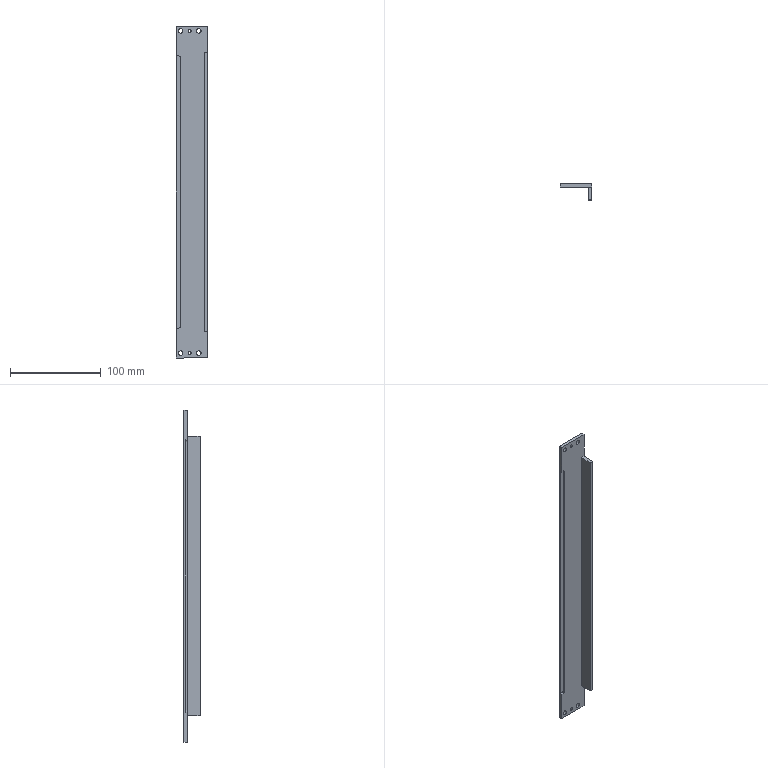Component | SolidWorks | CTM-HVS-52-OA-02-14-1 | 1 solid | 28 faces | box 35 x 18 x 366 mm | volume 65111 mm3 | cylinder 14 | plane 14 | commonest cylinder face diameters 5 x10 3.3 x4 | material 316L
build123d program:
from build123d import *

# Parameters (mm, degrees)
SKETCH1_W                  = 366
SKETCH1_H                  = 35
EXTRUDE1_DEPTH             = 4
SKETCH2_W                  = 308
SKETCH2_H                  = 4
EXTRUDE2_DEPTH             = 14
SKETCH4_W                  = 300
SKETCH4_H                  = 5
CUT_EXTRUDE1_DEPTH         = 2
FILLET1_R                  = 2.5
M6_TAPPED_HOLE1_AT_2_COUNT = 2
M6_TAPPED_HOLE1_AT_2_PITCH = 20


with BuildPart() as part:
    # Sketch1 → Extrude1 (new body)
    with BuildSketch(Plane.XY):
        Rectangle(SKETCH1_W, SKETCH1_H)
    extrude(amount=EXTRUDE1_DEPTH)

    # Sketch2 → Extrude2 (add)
    with BuildSketch(Plane.XY.offset(4)):
        with Locations((0, -15.5)):
            Rectangle(SKETCH2_W, SKETCH2_H)
    extrude(amount=EXTRUDE2_DEPTH)

    # Sketch4 → Cut-Extrude1 (cut)
    with BuildSketch(Plane.XY.offset(4)):
        with Locations((0, 15)):
            Rectangle(SKETCH4_W, SKETCH4_H)
    extrude(amount=-CUT_EXTRUDE1_DEPTH, mode=Mode.SUBTRACT)

    # Fillet1
    fillet1_edges = [part.edges().sort_by_distance(p)[0] for p in [
        (-150, 12.5, 3),
        (150, 12.5, 3),
    ]]
    fillet(fillet1_edges, radius=FILLET1_R)

    # Sketch5 → M6 Tapped Hole1 (revolve, cut)
    with BuildSketch(Plane(origin=(-177.5, 12.5, 4), x_dir=(0, -1, 0), z_dir=(1, 0, 0))):
        Polygon((0, 0), (0, 18.502), (2.5, 17), (2.5, 0), align=None)
    m6_tapped_hole1 = revolve(axis=Axis((-177.5, 12.5, 10.35), (0, 0, -1)), mode=Mode.SUBTRACT)

    # M6 Tapped Hole1 at 2: M6 Tapped Hole1 ×2
    with Locations(*[(0, -i * M6_TAPPED_HOLE1_AT_2_PITCH, 0) for i in range(1, M6_TAPPED_HOLE1_AT_2_COUNT)]):
        add(m6_tapped_hole1, mode=Mode.SUBTRACT)

    # Sketch7 → M4 Tapped Hole1 (revolve, cut)
    with BuildSketch(Plane(origin=(-177.5, 2.5, 4), x_dir=(0, -1, 0), z_dir=(1, 0, 0))):
        Polygon((0, 0), (0, 12.491), (1.65, 11.5), (1.65, 0), align=None)
    m4_tapped_hole1 = revolve(axis=Axis((-177.5, 2.5, 10.35), (0, 0, -1)), mode=Mode.SUBTRACT)

    # Mirror1: M6 Tapped Hole1, M4 Tapped Hole1 across plane
    add(m6_tapped_hole1.mirror(Plane(origin=(0, 0, 0), x_dir=(0, 0, 1), z_dir=(1, 0, 0))), mode=Mode.SUBTRACT)
    add(m4_tapped_hole1.mirror(Plane(origin=(0, 0, 0), x_dir=(0, 0, 1), z_dir=(1, 0, 0))), mode=Mode.SUBTRACT)

    # Mirror1 copy 1 sketch → Mirror1 copy 1 (revolve, cut)
    with BuildSketch(Plane(origin=(177.5, -7.5, 4), x_dir=(0, -1, 0), z_dir=(-1, 0, 0))):
        Polygon((0, 0), (0, -18.502), (2.5, -17), (2.5, 0), align=None)
    revolve(axis=Axis((177.5, -7.5, 10.35), (0, 0, 1)), mode=Mode.SUBTRACT)


solid = part.part

# Placed as in the assembly
solid = solid.moved(Location((292.693, -60.557, 192.5), (90, 0, 90)))
STEP:
#1=COLOUR_RGB('',0.7922,0.8196,0.9333);
#2=FILL_AREA_STYLE_COLOUR('',#1);
#3=FILL_AREA_STYLE('',(#2));
#4=SURFACE_STYLE_FILL_AREA(#3);
#5=SURFACE_SIDE_STYLE('',(#4));
#6=SURFACE_STYLE_USAGE(.BOTH.,#5);
#7=PRESENTATION_STYLE_ASSIGNMENT((#6));
#8=CARTESIAN_POINT('',(11.425,-2.384,14.502));
#9=VERTEX_POINT('',#8);
#10=CARTESIAN_POINT('',(11.425,-2.384,14.632));
#11=VERTEX_POINT('',#10);
#12=CARTESIAN_POINT('',(11.425,-2.384,14.567));
#13=DIRECTION('',(-0.,-1.,-0.));
#14=DIRECTION('',(0.,0.,1.));
#15=AXIS2_PLACEMENT_3D('',#12,#13,#14);
#16=CIRCLE('',#15,0.06496);
#17=EDGE_CURVE('',#9,#11,#16,.T.);
#18=ORIENTED_EDGE('',*,*,#17,.F.);
#19=CARTESIAN_POINT('',(11.425,-2.542,14.502));
#20=VERTEX_POINT('',#19);
#21=CARTESIAN_POINT('',(11.425,-2.542,14.502));
#22=DIRECTION('',(-0.,-1.,-0.));
#23=VECTOR('',#22,39.37);
#24=LINE('',#21,#23);
#25=EDGE_CURVE('',#9,#20,#24,.T.);
#26=ORIENTED_EDGE('',*,*,#25,.T.);
#27=CARTESIAN_POINT('',(11.425,-2.542,14.632));
#28=VERTEX_POINT('',#27);
#29=CARTESIAN_POINT('',(11.425,-2.542,14.567));
#30=DIRECTION('',(-0.,-1.,-0.));
#31=DIRECTION('',(0.,0.,1.));
#32=AXIS2_PLACEMENT_3D('',#29,#30,#31);
#33=CIRCLE('',#32,0.06496);
#34=EDGE_CURVE('',#20,#28,#33,.T.);
#35=ORIENTED_EDGE('',*,*,#34,.T.);
#36=CARTESIAN_POINT('',(11.425,-2.542,14.632));
#37=DIRECTION('',(-0.,-1.,-0.));
#38=VECTOR('',#37,39.37);
#39=LINE('',#36,#38);
#40=EDGE_CURVE('',#11,#28,#39,.T.);
#41=ORIENTED_EDGE('',*,*,#40,.F.);
#42=EDGE_LOOP('',(#18,#26,#35,#41));
#43=FACE_OUTER_BOUND('',#42,.T.);
#44=CARTESIAN_POINT('',(11.425,-2.542,14.567));
#45=DIRECTION('',(-0.,-1.,-0.));
#46=DIRECTION('',(0.,0.,1.));
#47=AXIS2_PLACEMENT_3D('',#44,#45,#46);
#48=CYLINDRICAL_SURFACE('',#47,0.06496);
#49=ADVANCED_FACE('',(#43),#48,.F.);
#50=CARTESIAN_POINT('',(11.031,-2.384,14.469));
#51=VERTEX_POINT('',#50);
#52=CARTESIAN_POINT('',(11.031,-2.384,14.665));
#53=VERTEX_POINT('',#52);
#54=CARTESIAN_POINT('',(11.031,-2.384,14.567));
#55=DIRECTION('',(-0.,-1.,-0.));
#56=DIRECTION('',(0.,0.,1.));
#57=AXIS2_PLACEMENT_3D('',#54,#55,#56);
#58=CIRCLE('',#57,0.09843);
#59=EDGE_CURVE('',#51,#53,#58,.T.);
#60=ORIENTED_EDGE('',*,*,#59,.F.);
#61=CARTESIAN_POINT('',(11.031,-2.542,14.469));
#62=VERTEX_POINT('',#61);
#63=CARTESIAN_POINT('',(11.031,-2.542,14.469));
#64=DIRECTION('',(-0.,-1.,-0.));
#65=VECTOR('',#64,39.37);
#66=LINE('',#63,#65);
#67=EDGE_CURVE('',#51,#62,#66,.T.);
#68=ORIENTED_EDGE('',*,*,#67,.T.);
#69=CARTESIAN_POINT('',(11.031,-2.542,14.665));
#70=VERTEX_POINT('',#69);
#71=CARTESIAN_POINT('',(11.031,-2.542,14.567));
#72=DIRECTION('',(-0.,-1.,-0.));
#73=DIRECTION('',(0.,0.,1.));
#74=AXIS2_PLACEMENT_3D('',#71,#72,#73);
#75=CIRCLE('',#74,0.09843);
#76=EDGE_CURVE('',#62,#70,#75,.T.);
#77=ORIENTED_EDGE('',*,*,#76,.T.);
#78=CARTESIAN_POINT('',(11.031,-2.542,14.665));
#79=DIRECTION('',(-0.,-1.,-0.));
#80=VECTOR('',#79,39.37);
#81=LINE('',#78,#80);
#82=EDGE_CURVE('',#53,#70,#81,.T.);
#83=ORIENTED_EDGE('',*,*,#82,.F.);
#84=EDGE_LOOP('',(#60,#68,#77,#83));
#85=FACE_OUTER_BOUND('',#84,.T.);
#86=CARTESIAN_POINT('',(11.031,-2.542,14.567));
#87=DIRECTION('',(-0.,-1.,-0.));
#88=DIRECTION('',(0.,0.,1.));
#89=AXIS2_PLACEMENT_3D('',#86,#87,#88);
#90=CYLINDRICAL_SURFACE('',#89,0.09843);
#91=ADVANCED_FACE('',(#85),#90,.F.);
#92=CARTESIAN_POINT('',(11.819,-2.384,14.469));
#93=VERTEX_POINT('',#92);
#94=CARTESIAN_POINT('',(11.819,-2.384,14.665));
#95=VERTEX_POINT('',#94);
#96=CARTESIAN_POINT('',(11.819,-2.384,14.567));
#97=DIRECTION('',(-0.,-1.,-0.));
#98=DIRECTION('',(0.,0.,1.));
#99=AXIS2_PLACEMENT_3D('',#96,#97,#98);
#100=CIRCLE('',#99,0.09843);
#101=EDGE_CURVE('',#93,#95,#100,.T.);
#102=ORIENTED_EDGE('',*,*,#101,.F.);
#103=CARTESIAN_POINT('',(11.819,-2.542,14.469));
#104=VERTEX_POINT('',#103);
#105=CARTESIAN_POINT('',(11.819,-2.542,14.469));
#106=DIRECTION('',(-0.,-1.,-0.));
#107=VECTOR('',#106,39.37);
#108=LINE('',#105,#107);
#109=EDGE_CURVE('',#93,#104,#108,.T.);
#110=ORIENTED_EDGE('',*,*,#109,.T.);
#111=CARTESIAN_POINT('',(11.819,-2.542,14.665));
#112=VERTEX_POINT('',#111);
#113=CARTESIAN_POINT('',(11.819,-2.542,14.567));
#114=DIRECTION('',(-0.,-1.,-0.));
#115=DIRECTION('',(0.,0.,1.));
#116=AXIS2_PLACEMENT_3D('',#113,#114,#115);
#117=CIRCLE('',#116,0.09843);
#118=EDGE_CURVE('',#104,#112,#117,.T.);
#119=ORIENTED_EDGE('',*,*,#118,.T.);
#120=CARTESIAN_POINT('',(11.819,-2.542,14.665));
#121=DIRECTION('',(-0.,-1.,-0.));
#122=VECTOR('',#121,39.37);
#123=LINE('',#120,#122);
#124=EDGE_CURVE('',#95,#112,#123,.T.);
#125=ORIENTED_EDGE('',*,*,#124,.F.);
#126=EDGE_LOOP('',(#102,#110,#119,#125));
#127=FACE_OUTER_BOUND('',#126,.T.);
#128=CARTESIAN_POINT('',(11.819,-2.542,14.567));
#129=DIRECTION('',(-0.,-1.,-0.));
#130=DIRECTION('',(0.,0.,1.));
#131=AXIS2_PLACEMENT_3D('',#128,#129,#130);
#132=CYLINDRICAL_SURFACE('',#131,0.09843);
#133=ADVANCED_FACE('',(#127),#132,.F.);
#134=CARTESIAN_POINT('',(11.425,-2.384,0.5256));
#135=VERTEX_POINT('',#134);
#136=CARTESIAN_POINT('',(11.425,-2.384,0.6555));
#137=VERTEX_POINT('',#136);
#138=CARTESIAN_POINT('',(11.425,-2.384,0.5906));
#139=DIRECTION('',(-0.,-1.,-0.));
#140=DIRECTION('',(0.,0.,1.));
#141=AXIS2_PLACEMENT_3D('',#138,#139,#140);
#142=CIRCLE('',#141,0.06496);
#143=EDGE_CURVE('',#135,#137,#142,.T.);
#144=ORIENTED_EDGE('',*,*,#143,.F.);
#145=CARTESIAN_POINT('',(11.425,-2.542,0.5256));
#146=VERTEX_POINT('',#145);
#147=CARTESIAN_POINT('',(11.425,-2.542,0.5256));
#148=DIRECTION('',(-0.,-1.,-0.));
#149=VECTOR('',#148,39.37);
#150=LINE('',#147,#149);
#151=EDGE_CURVE('',#135,#146,#150,.T.);
#152=ORIENTED_EDGE('',*,*,#151,.T.);
#153=CARTESIAN_POINT('',(11.425,-2.542,0.6555));
#154=VERTEX_POINT('',#153);
#155=CARTESIAN_POINT('',(11.425,-2.542,0.5906));
#156=DIRECTION('',(-0.,-1.,-0.));
#157=DIRECTION('',(0.,0.,1.));
#158=AXIS2_PLACEMENT_3D('',#155,#156,#157);
#159=CIRCLE('',#158,0.06496);
#160=EDGE_CURVE('',#146,#154,#159,.T.);
#161=ORIENTED_EDGE('',*,*,#160,.T.);
#162=CARTESIAN_POINT('',(11.425,-2.542,0.6555));
#163=DIRECTION('',(-0.,-1.,-0.));
#164=VECTOR('',#163,39.37);
#165=LINE('',#162,#164);
#166=EDGE_CURVE('',#137,#154,#165,.T.);
#167=ORIENTED_EDGE('',*,*,#166,.F.);
#168=EDGE_LOOP('',(#144,#152,#161,#167));
#169=FACE_OUTER_BOUND('',#168,.T.);
#170=CARTESIAN_POINT('',(11.425,-2.542,0.5906));
#171=DIRECTION('',(-0.,-1.,-0.));
#172=DIRECTION('',(0.,0.,1.));
#173=AXIS2_PLACEMENT_3D('',#170,#171,#172);
#174=CYLINDRICAL_SURFACE('',#173,0.06496);
#175=ADVANCED_FACE('',(#169),#174,.F.);
#176=CARTESIAN_POINT('',(11.031,-2.384,0.4921));
#177=VERTEX_POINT('',#176);
#178=CARTESIAN_POINT('',(11.031,-2.384,0.689));
#179=VERTEX_POINT('',#178);
#180=CARTESIAN_POINT('',(11.031,-2.384,0.5906));
#181=DIRECTION('',(-0.,-1.,-0.));
#182=DIRECTION('',(0.,0.,1.));
#183=AXIS2_PLACEMENT_3D('',#180,#181,#182);
#184=CIRCLE('',#183,0.09843);
#185=EDGE_CURVE('',#177,#179,#184,.T.);
#186=ORIENTED_EDGE('',*,*,#185,.F.);
#187=CARTESIAN_POINT('',(11.031,-2.542,0.4921));
#188=VERTEX_POINT('',#187);
#189=CARTESIAN_POINT('',(11.031,-2.542,0.4921));
#190=DIRECTION('',(-0.,-1.,-0.));
#191=VECTOR('',#190,39.37);
#192=LINE('',#189,#191);
#193=EDGE_CURVE('',#177,#188,#192,.T.);
#194=ORIENTED_EDGE('',*,*,#193,.T.);
#195=CARTESIAN_POINT('',(11.031,-2.542,0.689));
#196=VERTEX_POINT('',#195);
#197=CARTESIAN_POINT('',(11.031,-2.542,0.5906));
#198=DIRECTION('',(-0.,-1.,-0.));
#199=DIRECTION('',(0.,0.,1.));
#200=AXIS2_PLACEMENT_3D('',#197,#198,#199);
#201=CIRCLE('',#200,0.09843);
#202=EDGE_CURVE('',#188,#196,#201,.T.);
#203=ORIENTED_EDGE('',*,*,#202,.T.);
#204=CARTESIAN_POINT('',(11.031,-2.542,0.689));
#205=DIRECTION('',(-0.,-1.,-0.));
#206=VECTOR('',#205,39.37);
#207=LINE('',#204,#206);
#208=EDGE_CURVE('',#179,#196,#207,.T.);
#209=ORIENTED_EDGE('',*,*,#208,.F.);
#210=EDGE_LOOP('',(#186,#194,#203,#209));
#211=FACE_OUTER_BOUND('',#210,.T.);
#212=CARTESIAN_POINT('',(11.031,-2.542,0.5906));
#213=DIRECTION('',(-0.,-1.,-0.));
#214=DIRECTION('',(0.,0.,1.));
#215=AXIS2_PLACEMENT_3D('',#212,#213,#214);
#216=CYLINDRICAL_SURFACE('',#215,0.09843);
#217=ADVANCED_FACE('',(#211),#216,.F.);
#218=CARTESIAN_POINT('',(11.819,-2.384,0.4921));
#219=VERTEX_POINT('',#218);
#220=CARTESIAN_POINT('',(11.819,-2.384,0.689));
#221=VERTEX_POINT('',#220);
#222=CARTESIAN_POINT('',(11.819,-2.384,0.5906));
#223=DIRECTION('',(-0.,-1.,-0.));
#224=DIRECTION('',(0.,0.,1.));
#225=AXIS2_PLACEMENT_3D('',#222,#223,#224);
#226=CIRCLE('',#225,0.09843);
#227=EDGE_CURVE('',#219,#221,#226,.T.);
#228=ORIENTED_EDGE('',*,*,#227,.F.);
#229=CARTESIAN_POINT('',(11.819,-2.542,0.4921));
#230=VERTEX_POINT('',#229);
#231=CARTESIAN_POINT('',(11.819,-2.542,0.4921));
#232=DIRECTION('',(-0.,-1.,-0.));
#233=VECTOR('',#232,39.37);
#234=LINE('',#231,#233);
#235=EDGE_CURVE('',#219,#230,#234,.T.);
#236=ORIENTED_EDGE('',*,*,#235,.T.);
#237=CARTESIAN_POINT('',(11.819,-2.542,0.689));
#238=VERTEX_POINT('',#237);
#239=CARTESIAN_POINT('',(11.819,-2.542,0.5906));
#240=DIRECTION('',(-0.,-1.,-0.));
#241=DIRECTION('',(0.,0.,1.));
#242=AXIS2_PLACEMENT_3D('',#239,#240,#241);
#243=CIRCLE('',#242,0.09843);
#244=EDGE_CURVE('',#230,#238,#243,.T.);
#245=ORIENTED_EDGE('',*,*,#244,.T.);
#246=CARTESIAN_POINT('',(11.819,-2.542,0.689));
#247=DIRECTION('',(-0.,-1.,-0.));
#248=VECTOR('',#247,39.37);
#249=LINE('',#246,#248);
#250=EDGE_CURVE('',#221,#238,#249,.T.);
#251=ORIENTED_EDGE('',*,*,#250,.F.);
#252=EDGE_LOOP('',(#228,#236,#245,#251));
#253=FACE_OUTER_BOUND('',#252,.T.);
#254=CARTESIAN_POINT('',(11.819,-2.542,0.5906));
#255=DIRECTION('',(-0.,-1.,-0.));
#256=DIRECTION('',(0.,0.,1.));
#257=AXIS2_PLACEMENT_3D('',#254,#255,#256);
#258=CYLINDRICAL_SURFACE('',#257,0.09843);
#259=ADVANCED_FACE('',(#253),#258,.F.);
#260=CARTESIAN_POINT('',(12.212,-2.384,14.783));
#261=VERTEX_POINT('',#260);
#262=CARTESIAN_POINT('',(10.834,-2.384,14.783));
#263=VERTEX_POINT('',#262);
#264=CARTESIAN_POINT('',(10.834,-2.384,14.783));
#265=DIRECTION('',(-1.,0.,-0.));
#266=VECTOR('',#265,39.37);
#267=LINE('',#264,#266);
#268=EDGE_CURVE('',#261,#263,#267,.T.);
#269=ORIENTED_EDGE('',*,*,#268,.T.);
#270=CARTESIAN_POINT('',(10.834,-2.542,14.783));
#271=VERTEX_POINT('',#270);
#272=CARTESIAN_POINT('',(10.834,-2.542,14.783));
#273=DIRECTION('',(0.,1.,0.));
#274=VECTOR('',#273,39.37);
#275=LINE('',#272,#274);
#276=EDGE_CURVE('',#271,#263,#275,.T.);
#277=ORIENTED_EDGE('',*,*,#276,.F.);
#278=CARTESIAN_POINT('',(12.212,-2.542,14.783));
#279=VERTEX_POINT('',#278);
#280=CARTESIAN_POINT('',(10.834,-2.542,14.783));
#281=DIRECTION('',(-1.,0.,-0.));
#282=VECTOR('',#281,39.37);
#283=LINE('',#280,#282);
#284=EDGE_CURVE('',#279,#271,#283,.T.);
#285=ORIENTED_EDGE('',*,*,#284,.F.);
#286=CARTESIAN_POINT('',(12.212,-2.542,14.783));
#287=DIRECTION('',(0.,1.,0.));
#288=VECTOR('',#287,39.37);
#289=LINE('',#286,#288);
#290=EDGE_CURVE('',#279,#261,#289,.T.);
#291=ORIENTED_EDGE('',*,*,#290,.T.);
#292=EDGE_LOOP('',(#269,#277,#285,#291));
#293=FACE_OUTER_BOUND('',#292,.T.);
#294=CARTESIAN_POINT('',(10.834,-2.542,14.783));
#295=DIRECTION('',(0.,0.,-1.));
#296=DIRECTION('',(-0.,-1.,-0.));
#297=AXIS2_PLACEMENT_3D('',#294,#295,#296);
#298=PLANE('',#297);
#299=ADVANCED_FACE('',(#293),#298,.F.);
#300=CARTESIAN_POINT('',(10.834,-2.542,1.673));
#301=VERTEX_POINT('',#300);
#302=CARTESIAN_POINT('',(10.834,-2.542,0.374));
#303=VERTEX_POINT('',#302);
#304=CARTESIAN_POINT('',(10.834,-2.542,0.374));
#305=DIRECTION('',(0.,-0.,-1.));
#306=VECTOR('',#305,39.37);
#307=LINE('',#304,#306);
#308=EDGE_CURVE('',#301,#303,#307,.T.);
#309=ORIENTED_EDGE('',*,*,#308,.F.);
#310=CARTESIAN_POINT('',(10.834,-2.463,1.673));
#311=VERTEX_POINT('',#310);
#312=CARTESIAN_POINT('',(10.834,-2.463,1.673));
#313=DIRECTION('',(-0.,-1.,-0.));
#314=VECTOR('',#313,39.37);
#315=LINE('',#312,#314);
#316=EDGE_CURVE('',#311,#301,#315,.T.);
#317=ORIENTED_EDGE('',*,*,#316,.F.);
#318=CARTESIAN_POINT('',(10.834,-2.463,13.484));
#319=VERTEX_POINT('',#318);
#320=CARTESIAN_POINT('',(10.834,-2.463,13.484));
#321=DIRECTION('',(0.,-0.,-1.));
#322=VECTOR('',#321,39.37);
#323=LINE('',#320,#322);
#324=EDGE_CURVE('',#319,#311,#323,.T.);
#325=ORIENTED_EDGE('',*,*,#324,.F.);
#326=CARTESIAN_POINT('',(10.834,-2.542,13.484));
#327=VERTEX_POINT('',#326);
#328=CARTESIAN_POINT('',(10.834,-2.463,13.484));
#329=DIRECTION('',(-0.,-1.,-0.));
#330=VECTOR('',#329,39.37);
#331=LINE('',#328,#330);
#332=EDGE_CURVE('',#319,#327,#331,.T.);
#333=ORIENTED_EDGE('',*,*,#332,.T.);
#334=CARTESIAN_POINT('',(10.834,-2.542,0.374));
#335=DIRECTION('',(0.,-0.,-1.));
#336=VECTOR('',#335,39.37);
#337=LINE('',#334,#336);
#338=EDGE_CURVE('',#271,#327,#337,.T.);
#339=ORIENTED_EDGE('',*,*,#338,.F.);
#340=ORIENTED_EDGE('',*,*,#276,.T.);
#341=CARTESIAN_POINT('',(10.834,-2.384,0.374));
#342=VERTEX_POINT('',#341);
#343=CARTESIAN_POINT('',(10.834,-2.384,0.374));
#344=DIRECTION('',(0.,-0.,-1.));
#345=VECTOR('',#344,39.37);
#346=LINE('',#343,#345);
#347=EDGE_CURVE('',#263,#342,#346,.T.);
#348=ORIENTED_EDGE('',*,*,#347,.T.);
#349=CARTESIAN_POINT('',(10.834,-2.542,0.374));
#350=DIRECTION('',(0.,1.,0.));
#351=VECTOR('',#350,39.37);
#352=LINE('',#349,#351);
#353=EDGE_CURVE('',#303,#342,#352,.T.);
#354=ORIENTED_EDGE('',*,*,#353,.F.);
#355=EDGE_LOOP('',(#309,#317,#325,#333,#339,#340,#348,#354));
#356=FACE_OUTER_BOUND('',#355,.T.);
#357=CARTESIAN_POINT('',(10.834,-2.542,0.374));
#358=DIRECTION('',(1.,-0.,0.));
#359=DIRECTION('',(0.,1.,0.));
#360=AXIS2_PLACEMENT_3D('',#357,#358,#359);
#361=PLANE('',#360);
#362=ADVANCED_FACE('',(#356),#361,.F.);
#363=CARTESIAN_POINT('',(12.212,-2.384,0.374));
#364=VERTEX_POINT('',#363);
#365=CARTESIAN_POINT('',(10.834,-2.384,0.374));
#366=DIRECTION('',(1.,-0.,0.));
#367=VECTOR('',#366,39.37);
#368=LINE('',#365,#367);
#369=EDGE_CURVE('',#342,#364,#368,.T.);
#370=ORIENTED_EDGE('',*,*,#369,.T.);
#371=CARTESIAN_POINT('',(12.212,-2.542,0.374));
#372=VERTEX_POINT('',#371);
#373=CARTESIAN_POINT('',(12.212,-2.542,0.374));
#374=DIRECTION('',(0.,1.,0.));
#375=VECTOR('',#374,39.37);
#376=LINE('',#373,#375);
#377=EDGE_CURVE('',#372,#364,#376,.T.);
#378=ORIENTED_EDGE('',*,*,#377,.F.);
#379=CARTESIAN_POINT('',(10.834,-2.542,0.374));
#380=DIRECTION('',(1.,-0.,0.));
#381=VECTOR('',#380,39.37);
#382=LINE('',#379,#381);
#383=EDGE_CURVE('',#303,#372,#382,.T.);
#384=ORIENTED_EDGE('',*,*,#383,.F.);
#385=ORIENTED_EDGE('',*,*,#353,.T.);
#386=EDGE_LOOP('',(#370,#378,#384,#385));
#387=FACE_OUTER_BOUND('',#386,.T.);
#388=CARTESIAN_POINT('',(10.834,-2.542,0.374));
#389=DIRECTION('',(-0.,-0.,1.));
#390=DIRECTION('',(0.,1.,0.));
#391=AXIS2_PLACEMENT_3D('',#388,#389,#390);
#392=PLANE('',#391);
#393=ADVANCED_FACE('',(#387),#392,.F.);
#394=CARTESIAN_POINT('',(12.212,-2.384,0.374));
#395=DIRECTION('',(-0.,0.,1.));
#396=VECTOR('',#395,39.37);
#397=LINE('',#394,#396);
#398=EDGE_CURVE('',#364,#261,#397,.T.);
#399=ORIENTED_EDGE('',*,*,#398,.T.);
#400=ORIENTED_EDGE('',*,*,#290,.F.);
#401=CARTESIAN_POINT('',(12.212,-2.542,13.642));
#402=VERTEX_POINT('',#401);
#403=CARTESIAN_POINT('',(12.212,-2.542,0.374));
#404=DIRECTION('',(-0.,0.,1.));
#405=VECTOR('',#404,39.37);
#406=LINE('',#403,#405);
#407=EDGE_CURVE('',#402,#279,#406,.T.);
#408=ORIENTED_EDGE('',*,*,#407,.F.);
#409=CARTESIAN_POINT('',(12.212,-3.093,13.642));
#410=VERTEX_POINT('',#409);
#411=CARTESIAN_POINT('',(12.212,-3.093,13.642));
#412=DIRECTION('',(0.,1.,0.));
#413=VECTOR('',#412,39.37);
#414=LINE('',#411,#413);
#415=EDGE_CURVE('',#410,#402,#414,.T.);
#416=ORIENTED_EDGE('',*,*,#415,.F.);
#417=CARTESIAN_POINT('',(12.212,-3.093,1.516));
#418=VERTEX_POINT('',#417);
#419=CARTESIAN_POINT('',(12.212,-3.093,1.516));
#420=DIRECTION('',(-0.,0.,1.));
#421=VECTOR('',#420,39.37);
#422=LINE('',#419,#421);
#423=EDGE_CURVE('',#418,#410,#422,.T.);
#424=ORIENTED_EDGE('',*,*,#423,.F.);
#425=CARTESIAN_POINT('',(12.212,-2.542,1.516));
#426=VERTEX_POINT('',#425);
#427=CARTESIAN_POINT('',(12.212,-3.093,1.516));
#428=DIRECTION('',(0.,1.,0.));
#429=VECTOR('',#428,39.37);
#430=LINE('',#427,#429);
#431=EDGE_CURVE('',#418,#426,#430,.T.);
#432=ORIENTED_EDGE('',*,*,#431,.T.);
#433=CARTESIAN_POINT('',(12.212,-2.542,0.374));
#434=DIRECTION('',(-0.,0.,1.));
#435=VECTOR('',#434,39.37);
#436=LINE('',#433,#435);
#437=EDGE_CURVE('',#372,#426,#436,.T.);
#438=ORIENTED_EDGE('',*,*,#437,.F.);
#439=ORIENTED_EDGE('',*,*,#377,.T.);
#440=EDGE_LOOP('',(#399,#400,#408,#416,#424,#432,#438,#439));
#441=FACE_OUTER_BOUND('',#440,.T.);
#442=CARTESIAN_POINT('',(12.212,-2.542,0.374));
#443=DIRECTION('',(-1.,0.,-0.));
#444=DIRECTION('',(-0.,-1.,-0.));
#445=AXIS2_PLACEMENT_3D('',#442,#443,#444);
#446=PLANE('',#445);
#447=ADVANCED_FACE('',(#441),#446,.F.);
#448=CARTESIAN_POINT('',(11.425,-2.542,14.567));
#449=DIRECTION('',(-0.,-1.,-0.));
#450=DIRECTION('',(0.,0.,1.));
#451=AXIS2_PLACEMENT_3D('',#448,#449,#450);
#452=CIRCLE('',#451,0.06496);
#453=EDGE_CURVE('',#28,#20,#452,.T.);
#454=ORIENTED_EDGE('',*,*,#453,.F.);
#455=ORIENTED_EDGE('',*,*,#34,.F.);
#456=EDGE_LOOP('',(#454,#455));
#457=FACE_BOUND('',#456,.T.);
#458=CARTESIAN_POINT('',(11.031,-2.542,14.567));
#459=DIRECTION('',(-0.,-1.,-0.));
#460=DIRECTION('',(0.,0.,1.));
#461=AXIS2_PLACEMENT_3D('',#458,#459,#460);
#462=CIRCLE('',#461,0.09843);
#463=EDGE_CURVE('',#70,#62,#462,.T.);
#464=ORIENTED_EDGE('',*,*,#463,.F.);
#465=ORIENTED_EDGE('',*,*,#76,.F.);
#466=EDGE_LOOP('',(#464,#465));
#467=FACE_BOUND('',#466,.T.);
#468=CARTESIAN_POINT('',(11.819,-2.542,14.567));
#469=DIRECTION('',(-0.,-1.,-0.));
#470=DIRECTION('',(0.,0.,1.));
#471=AXIS2_PLACEMENT_3D('',#468,#469,#470);
#472=CIRCLE('',#471,0.09843);
#473=EDGE_CURVE('',#112,#104,#472,.T.);
#474=ORIENTED_EDGE('',*,*,#473,.F.);
#475=ORIENTED_EDGE('',*,*,#118,.F.);
#476=EDGE_LOOP('',(#474,#475));
#477=FACE_BOUND('',#476,.T.);
#478=CARTESIAN_POINT('',(11.425,-2.542,0.5906));
#479=DIRECTION('',(-0.,-1.,-0.));
#480=DIRECTION('',(0.,0.,1.));
#481=AXIS2_PLACEMENT_3D('',#478,#479,#480);
#482=CIRCLE('',#481,0.06496);
#483=EDGE_CURVE('',#154,#146,#482,.T.);
#484=ORIENTED_EDGE('',*,*,#483,.F.);
#485=ORIENTED_EDGE('',*,*,#160,.F.);
#486=EDGE_LOOP('',(#484,#485));
#487=FACE_BOUND('',#486,.T.);
#488=CARTESIAN_POINT('',(11.031,-2.542,0.5906));
#489=DIRECTION('',(-0.,-1.,-0.));
#490=DIRECTION('',(0.,0.,1.));
#491=AXIS2_PLACEMENT_3D('',#488,#489,#490);
#492=CIRCLE('',#491,0.09843);
#493=EDGE_CURVE('',#196,#188,#492,.T.);
#494=ORIENTED_EDGE('',*,*,#493,.F.);
#495=ORIENTED_EDGE('',*,*,#202,.F.);
#496=EDGE_LOOP('',(#494,#495));
#497=FACE_BOUND('',#496,.T.);
#498=CARTESIAN_POINT('',(11.819,-2.542,0.5906));
#499=DIRECTION('',(-0.,-1.,-0.));
#500=DIRECTION('',(0.,0.,1.));
#501=AXIS2_PLACEMENT_3D('',#498,#499,#500);
#502=CIRCLE('',#501,0.09843);
#503=EDGE_CURVE('',#238,#230,#502,.T.);
#504=ORIENTED_EDGE('',*,*,#503,.F.);
#505=ORIENTED_EDGE('',*,*,#244,.F.);
#506=EDGE_LOOP('',(#504,#505));
#507=FACE_BOUND('',#506,.T.);
#508=CARTESIAN_POINT('',(10.933,-2.542,1.673));
#509=VERTEX_POINT('',#508);
#510=CARTESIAN_POINT('',(11.031,-2.542,1.673));
#511=DIRECTION('',(1.,-0.,0.));
#512=VECTOR('',#511,39.37);
#513=LINE('',#510,#512);
#514=EDGE_CURVE('',#301,#509,#513,.T.);
#515=ORIENTED_EDGE('',*,*,#514,.F.);
#516=ORIENTED_EDGE('',*,*,#308,.T.);
#517=ORIENTED_EDGE('',*,*,#383,.T.);
#518=ORIENTED_EDGE('',*,*,#437,.T.);
#519=CARTESIAN_POINT('',(12.055,-2.542,1.516));
#520=VERTEX_POINT('',#519);
#521=CARTESIAN_POINT('',(12.055,-2.542,1.516));
#522=DIRECTION('',(1.,-0.,0.));
#523=VECTOR('',#522,39.37);
#524=LINE('',#521,#523);
#525=EDGE_CURVE('',#520,#426,#524,.T.);
#526=ORIENTED_EDGE('',*,*,#525,.F.);
#527=CARTESIAN_POINT('',(12.055,-2.542,13.642));
#528=VERTEX_POINT('',#527);
#529=CARTESIAN_POINT('',(12.055,-2.542,1.516));
#530=DIRECTION('',(0.,-0.,-1.));
#531=VECTOR('',#530,39.37);
#532=LINE('',#529,#531);
#533=EDGE_CURVE('',#528,#520,#532,.T.);
#534=ORIENTED_EDGE('',*,*,#533,.F.);
#535=CARTESIAN_POINT('',(12.055,-2.542,13.642));
#536=DIRECTION('',(-1.,0.,-0.));
#537=VECTOR('',#536,39.37);
#538=LINE('',#535,#537);
#539=EDGE_CURVE('',#402,#528,#538,.T.);
#540=ORIENTED_EDGE('',*,*,#539,.F.);
#541=ORIENTED_EDGE('',*,*,#407,.T.);
#542=ORIENTED_EDGE('',*,*,#284,.T.);
#543=ORIENTED_EDGE('',*,*,#338,.T.);
#544=CARTESIAN_POINT('',(10.933,-2.542,13.484));
#545=VERTEX_POINT('',#544);
#546=CARTESIAN_POINT('',(11.031,-2.542,13.484));
#547=DIRECTION('',(-1.,0.,-0.));
#548=VECTOR('',#547,39.37);
#549=LINE('',#546,#548);
#550=EDGE_CURVE('',#545,#327,#549,.T.);
#551=ORIENTED_EDGE('',*,*,#550,.F.);
#552=CARTESIAN_POINT('',(11.031,-2.542,13.386));
#553=VERTEX_POINT('',#552);
#554=CARTESIAN_POINT('',(10.933,-2.542,13.386));
#555=DIRECTION('',(0.,1.,0.));
#556=DIRECTION('',(0.,0.,1.));
#557=AXIS2_PLACEMENT_3D('',#554,#555,#556);
#558=CIRCLE('',#557,0.09843);
#559=EDGE_CURVE('',#545,#553,#558,.T.);
#560=ORIENTED_EDGE('',*,*,#559,.T.);
#561=CARTESIAN_POINT('',(11.031,-2.542,1.772));
#562=VERTEX_POINT('',#561);
#563=CARTESIAN_POINT('',(11.031,-2.542,13.484));
#564=DIRECTION('',(-0.,0.,1.));
#565=VECTOR('',#564,39.37);
#566=LINE('',#563,#565);
#567=EDGE_CURVE('',#562,#553,#566,.T.);
#568=ORIENTED_EDGE('',*,*,#567,.F.);
#569=CARTESIAN_POINT('',(10.933,-2.542,1.772));
#570=DIRECTION('',(0.,1.,0.));
#571=DIRECTION('',(0.,0.,1.));
#572=AXIS2_PLACEMENT_3D('',#569,#570,#571);
#573=CIRCLE('',#572,0.09843);
#574=EDGE_CURVE('',#562,#509,#573,.T.);
#575=ORIENTED_EDGE('',*,*,#574,.T.);
#576=EDGE_LOOP('',(#515,#516,#517,#518,#526,#534,#540,#541,#542,#543,#551,#560,#568,#575));
#577=FACE_OUTER_BOUND('',#576,.T.);
#578=CARTESIAN_POINT('',(12.212,-2.542,14.783));
#579=DIRECTION('',(-0.,-1.,-0.));
#580=DIRECTION('',(-0.,0.,1.));
#581=AXIS2_PLACEMENT_3D('',#578,#579,#580);
#582=PLANE('',#581);
#583=ADVANCED_FACE('',(#457,#467,#477,#487,#497,#507,#577),#582,.T.);
#584=CARTESIAN_POINT('',(11.425,-2.384,14.567));
#585=DIRECTION('',(-0.,-1.,-0.));
#586=DIRECTION('',(0.,0.,1.));
#587=AXIS2_PLACEMENT_3D('',#584,#585,#586);
#588=CIRCLE('',#587,0.06496);
#589=EDGE_CURVE('',#11,#9,#588,.T.);
#590=ORIENTED_EDGE('',*,*,#589,.T.);
#591=ORIENTED_EDGE('',*,*,#17,.T.);
#592=EDGE_LOOP('',(#590,#591));
#593=FACE_BOUND('',#592,.T.);
#594=CARTESIAN_POINT('',(11.031,-2.384,14.567));
#595=DIRECTION('',(-0.,-1.,-0.));
#596=DIRECTION('',(0.,0.,1.));
#597=AXIS2_PLACEMENT_3D('',#594,#595,#596);
#598=CIRCLE('',#597,0.09843);
#599=EDGE_CURVE('',#53,#51,#598,.T.);
#600=ORIENTED_EDGE('',*,*,#599,.T.);
#601=ORIENTED_EDGE('',*,*,#59,.T.);
#602=EDGE_LOOP('',(#600,#601));
#603=FACE_BOUND('',#602,.T.);
#604=CARTESIAN_POINT('',(11.819,-2.384,14.567));
#605=DIRECTION('',(-0.,-1.,-0.));
#606=DIRECTION('',(0.,0.,1.));
#607=AXIS2_PLACEMENT_3D('',#604,#605,#606);
#608=CIRCLE('',#607,0.09843);
#609=EDGE_CURVE('',#95,#93,#608,.T.);
#610=ORIENTED_EDGE('',*,*,#609,.T.);
#611=ORIENTED_EDGE('',*,*,#101,.T.);
#612=EDGE_LOOP('',(#610,#611));
#613=FACE_BOUND('',#612,.T.);
#614=CARTESIAN_POINT('',(11.425,-2.384,0.5906));
#615=DIRECTION('',(-0.,-1.,-0.));
#616=DIRECTION('',(0.,0.,1.));
#617=AXIS2_PLACEMENT_3D('',#614,#615,#616);
#618=CIRCLE('',#617,0.06496);
#619=EDGE_CURVE('',#137,#135,#618,.T.);
#620=ORIENTED_EDGE('',*,*,#619,.T.);
#621=ORIENTED_EDGE('',*,*,#143,.T.);
#622=EDGE_LOOP('',(#620,#621));
#623=FACE_BOUND('',#622,.T.);
#624=CARTESIAN_POINT('',(11.031,-2.384,0.5906));
#625=DIRECTION('',(-0.,-1.,-0.));
#626=DIRECTION('',(0.,0.,1.));
#627=AXIS2_PLACEMENT_3D('',#624,#625,#626);
#628=CIRCLE('',#627,0.09843);
#629=EDGE_CURVE('',#179,#177,#628,.T.);
#630=ORIENTED_EDGE('',*,*,#629,.T.);
#631=ORIENTED_EDGE('',*,*,#185,.T.);
#632=EDGE_LOOP('',(#630,#631));
#633=FACE_BOUND('',#632,.T.);
#634=CARTESIAN_POINT('',(11.819,-2.384,0.5906));
#635=DIRECTION('',(-0.,-1.,-0.));
#636=DIRECTION('',(0.,0.,1.));
#637=AXIS2_PLACEMENT_3D('',#634,#635,#636);
#638=CIRCLE('',#637,0.09843);
#639=EDGE_CURVE('',#221,#219,#638,.T.);
#640=ORIENTED_EDGE('',*,*,#639,.T.);
#641=ORIENTED_EDGE('',*,*,#227,.T.);
#642=EDGE_LOOP('',(#640,#641));
#643=FACE_BOUND('',#642,.T.);
#644=ORIENTED_EDGE('',*,*,#268,.F.);
#645=ORIENTED_EDGE('',*,*,#398,.F.);
#646=ORIENTED_EDGE('',*,*,#369,.F.);
#647=ORIENTED_EDGE('',*,*,#347,.F.);
#648=EDGE_LOOP('',(#644,#645,#646,#647));
#649=FACE_OUTER_BOUND('',#648,.T.);
#650=CARTESIAN_POINT('',(12.212,-2.384,14.783));
#651=DIRECTION('',(-0.,-1.,-0.));
#652=DIRECTION('',(-0.,0.,1.));
#653=AXIS2_PLACEMENT_3D('',#650,#651,#652);
#654=PLANE('',#653);
#655=ADVANCED_FACE('',(#593,#603,#613,#623,#633,#643,#649),#654,.F.);
#656=ORIENTED_EDGE('',*,*,#539,.T.);
#657=CARTESIAN_POINT('',(12.055,-3.093,13.642));
#658=VERTEX_POINT('',#657);
#659=CARTESIAN_POINT('',(12.055,-3.093,13.642));
#660=DIRECTION('',(0.,1.,0.));
#661=VECTOR('',#660,39.37);
#662=LINE('',#659,#661);
#663=EDGE_CURVE('',#658,#528,#662,.T.);
#664=ORIENTED_EDGE('',*,*,#663,.F.);
#665=CARTESIAN_POINT('',(12.055,-3.093,13.642));
#666=DIRECTION('',(-1.,0.,-0.));
#667=VECTOR('',#666,39.37);
#668=LINE('',#665,#667);
#669=EDGE_CURVE('',#410,#658,#668,.T.);
#670=ORIENTED_EDGE('',*,*,#669,.F.);
#671=ORIENTED_EDGE('',*,*,#415,.T.);
#672=EDGE_LOOP('',(#656,#664,#670,#671));
#673=FACE_OUTER_BOUND('',#672,.T.);
#674=CARTESIAN_POINT('',(12.055,-3.093,13.642));
#675=DIRECTION('',(0.,0.,-1.));
#676=DIRECTION('',(-0.,-1.,-0.));
#677=AXIS2_PLACEMENT_3D('',#674,#675,#676);
#678=PLANE('',#677);
#679=ADVANCED_FACE('',(#673),#678,.F.);
#680=ORIENTED_EDGE('',*,*,#533,.T.);
#681=CARTESIAN_POINT('',(12.055,-3.093,1.516));
#682=VERTEX_POINT('',#681);
#683=CARTESIAN_POINT('',(12.055,-3.093,1.516));
#684=DIRECTION('',(0.,1.,0.));
#685=VECTOR('',#684,39.37);
#686=LINE('',#683,#685);
#687=EDGE_CURVE('',#682,#520,#686,.T.);
#688=ORIENTED_EDGE('',*,*,#687,.F.);
#689=CARTESIAN_POINT('',(12.055,-3.093,1.516));
#690=DIRECTION('',(0.,-0.,-1.));
#691=VECTOR('',#690,39.37);
#692=LINE('',#689,#691);
#693=EDGE_CURVE('',#658,#682,#692,.T.);
#694=ORIENTED_EDGE('',*,*,#693,.F.);
#695=ORIENTED_EDGE('',*,*,#663,.T.);
#696=EDGE_LOOP('',(#680,#688,#694,#695));
#697=FACE_OUTER_BOUND('',#696,.T.);
#698=CARTESIAN_POINT('',(12.055,-3.093,1.516));
#699=DIRECTION('',(1.,-0.,0.));
#700=DIRECTION('',(0.,1.,0.));
#701=AXIS2_PLACEMENT_3D('',#698,#699,#700);
#702=PLANE('',#701);
#703=ADVANCED_FACE('',(#697),#702,.F.);
#704=ORIENTED_EDGE('',*,*,#525,.T.);
#705=ORIENTED_EDGE('',*,*,#431,.F.);
#706=CARTESIAN_POINT('',(12.055,-3.093,1.516));
#707=DIRECTION('',(1.,-0.,0.));
#708=VECTOR('',#707,39.37);
#709=LINE('',#706,#708);
#710=EDGE_CURVE('',#682,#418,#709,.T.);
#711=ORIENTED_EDGE('',*,*,#710,.F.);
#712=ORIENTED_EDGE('',*,*,#687,.T.);
#713=EDGE_LOOP('',(#704,#705,#711,#712));
#714=FACE_OUTER_BOUND('',#713,.T.);
#715=CARTESIAN_POINT('',(12.055,-3.093,1.516));
#716=DIRECTION('',(-0.,-0.,1.));
#717=DIRECTION('',(0.,1.,0.));
#718=AXIS2_PLACEMENT_3D('',#715,#716,#717);
#719=PLANE('',#718);
#720=ADVANCED_FACE('',(#714),#719,.F.);
#721=ORIENTED_EDGE('',*,*,#669,.T.);
#722=ORIENTED_EDGE('',*,*,#693,.T.);
#723=ORIENTED_EDGE('',*,*,#710,.T.);
#724=ORIENTED_EDGE('',*,*,#423,.T.);
#725=EDGE_LOOP('',(#721,#722,#723,#724));
#726=FACE_OUTER_BOUND('',#725,.T.);
#727=CARTESIAN_POINT('',(12.212,-3.093,13.642));
#728=DIRECTION('',(-0.,-1.,-0.));
#729=DIRECTION('',(-0.,0.,1.));
#730=AXIS2_PLACEMENT_3D('',#727,#728,#729);
#731=PLANE('',#730);
#732=ADVANCED_FACE('',(#726),#731,.T.);
#733=ORIENTED_EDGE('',*,*,#514,.T.);
#734=CARTESIAN_POINT('',(10.933,-2.463,1.673));
#735=VERTEX_POINT('',#734);
#736=CARTESIAN_POINT('',(10.933,-2.463,1.673));
#737=DIRECTION('',(0.,1.,0.));
#738=VECTOR('',#737,39.37);
#739=LINE('',#736,#738);
#740=EDGE_CURVE('',#509,#735,#739,.T.);
#741=ORIENTED_EDGE('',*,*,#740,.T.);
#742=CARTESIAN_POINT('',(11.031,-2.463,1.673));
#743=DIRECTION('',(1.,-0.,0.));
#744=VECTOR('',#743,39.37);
#745=LINE('',#742,#744);
#746=EDGE_CURVE('',#311,#735,#745,.T.);
#747=ORIENTED_EDGE('',*,*,#746,.F.);
#748=ORIENTED_EDGE('',*,*,#316,.T.);
#749=EDGE_LOOP('',(#733,#741,#747,#748));
#750=FACE_OUTER_BOUND('',#749,.T.);
#751=CARTESIAN_POINT('',(11.031,-2.463,1.673));
#752=DIRECTION('',(0.,0.,-1.));
#753=DIRECTION('',(-0.,-1.,-0.));
#754=AXIS2_PLACEMENT_3D('',#751,#752,#753);
#755=PLANE('',#754);
#756=ADVANCED_FACE('',(#750),#755,.F.);
#757=CARTESIAN_POINT('',(10.933,-2.463,13.484));
#758=VERTEX_POINT('',#757);
#759=CARTESIAN_POINT('',(11.031,-2.463,13.484));
#760=DIRECTION('',(-1.,0.,-0.));
#761=VECTOR('',#760,39.37);
#762=LINE('',#759,#761);
#763=EDGE_CURVE('',#758,#319,#762,.T.);
#764=ORIENTED_EDGE('',*,*,#763,.F.);
#765=CARTESIAN_POINT('',(10.933,-2.542,13.484));
#766=DIRECTION('',(-0.,-1.,-0.));
#767=VECTOR('',#766,39.37);
#768=LINE('',#765,#767);
#769=EDGE_CURVE('',#758,#545,#768,.T.);
#770=ORIENTED_EDGE('',*,*,#769,.T.);
#771=ORIENTED_EDGE('',*,*,#550,.T.);
#772=ORIENTED_EDGE('',*,*,#332,.F.);
#773=EDGE_LOOP('',(#764,#770,#771,#772));
#774=FACE_OUTER_BOUND('',#773,.T.);
#775=CARTESIAN_POINT('',(11.031,-2.463,13.484));
#776=DIRECTION('',(-0.,-0.,1.));
#777=DIRECTION('',(0.,1.,0.));
#778=AXIS2_PLACEMENT_3D('',#775,#776,#777);
#779=PLANE('',#778);
#780=ADVANCED_FACE('',(#774),#779,.F.);
#781=ORIENTED_EDGE('',*,*,#567,.T.);
#782=CARTESIAN_POINT('',(11.031,-2.463,13.386));
#783=VERTEX_POINT('',#782);
#784=CARTESIAN_POINT('',(11.031,-2.463,13.386));
#785=DIRECTION('',(0.,1.,0.));
#786=VECTOR('',#785,39.37);
#787=LINE('',#784,#786);
#788=EDGE_CURVE('',#553,#783,#787,.T.);
#789=ORIENTED_EDGE('',*,*,#788,.T.);
#790=CARTESIAN_POINT('',(11.031,-2.463,1.772));
#791=VERTEX_POINT('',#790);
#792=CARTESIAN_POINT('',(11.031,-2.463,13.484));
#793=DIRECTION('',(-0.,0.,1.));
#794=VECTOR('',#793,39.37);
#795=LINE('',#792,#794);
#796=EDGE_CURVE('',#791,#783,#795,.T.);
#797=ORIENTED_EDGE('',*,*,#796,.F.);
#798=CARTESIAN_POINT('',(11.031,-2.542,1.772));
#799=DIRECTION('',(-0.,-1.,-0.));
#800=VECTOR('',#799,39.37);
#801=LINE('',#798,#800);
#802=EDGE_CURVE('',#791,#562,#801,.T.);
#803=ORIENTED_EDGE('',*,*,#802,.T.);
#804=EDGE_LOOP('',(#781,#789,#797,#803));
#805=FACE_OUTER_BOUND('',#804,.T.);
#806=CARTESIAN_POINT('',(11.031,-2.463,13.484));
#807=DIRECTION('',(1.,-0.,0.));
#808=DIRECTION('',(-0.,0.,1.));
#809=AXIS2_PLACEMENT_3D('',#806,#807,#808);
#810=PLANE('',#809);
#811=ADVANCED_FACE('',(#805),#810,.F.);
#812=ORIENTED_EDGE('',*,*,#796,.T.);
#813=CARTESIAN_POINT('',(10.933,-2.463,13.386));
#814=DIRECTION('',(-0.,-1.,-0.));
#815=DIRECTION('',(0.,0.,1.));
#816=AXIS2_PLACEMENT_3D('',#813,#814,#815);
#817=CIRCLE('',#816,0.09843);
#818=EDGE_CURVE('',#783,#758,#817,.T.);
#819=ORIENTED_EDGE('',*,*,#818,.T.);
#820=ORIENTED_EDGE('',*,*,#763,.T.);
#821=ORIENTED_EDGE('',*,*,#324,.T.);
#822=ORIENTED_EDGE('',*,*,#746,.T.);
#823=CARTESIAN_POINT('',(10.933,-2.463,1.772));
#824=DIRECTION('',(-0.,-1.,-0.));
#825=DIRECTION('',(0.,0.,1.));
#826=AXIS2_PLACEMENT_3D('',#823,#824,#825);
#827=CIRCLE('',#826,0.09843);
#828=EDGE_CURVE('',#735,#791,#827,.T.);
#829=ORIENTED_EDGE('',*,*,#828,.T.);
#830=EDGE_LOOP('',(#812,#819,#820,#821,#822,#829));
#831=FACE_OUTER_BOUND('',#830,.T.);
#832=CARTESIAN_POINT('',(10.834,-2.463,1.673));
#833=DIRECTION('',(-0.,-1.,-0.));
#834=DIRECTION('',(-0.,0.,1.));
#835=AXIS2_PLACEMENT_3D('',#832,#833,#834);
#836=PLANE('',#835);
#837=ADVANCED_FACE('',(#831),#836,.T.);
#838=ORIENTED_EDGE('',*,*,#818,.F.);
#839=ORIENTED_EDGE('',*,*,#788,.F.);
#840=ORIENTED_EDGE('',*,*,#559,.F.);
#841=ORIENTED_EDGE('',*,*,#769,.F.);
#842=EDGE_LOOP('',(#838,#839,#840,#841));
#843=FACE_OUTER_BOUND('',#842,.T.);
#844=CARTESIAN_POINT('',(10.933,-2.463,13.386));
#845=DIRECTION('',(0.,1.,0.));
#846=DIRECTION('',(0.,0.,-1.));
#847=AXIS2_PLACEMENT_3D('',#844,#845,#846);
#848=CYLINDRICAL_SURFACE('',#847,0.09843);
#849=ADVANCED_FACE('',(#843),#848,.F.);
#850=ORIENTED_EDGE('',*,*,#828,.F.);
#851=ORIENTED_EDGE('',*,*,#740,.F.);
#852=ORIENTED_EDGE('',*,*,#574,.F.);
#853=ORIENTED_EDGE('',*,*,#802,.F.);
#854=EDGE_LOOP('',(#850,#851,#852,#853));
#855=FACE_OUTER_BOUND('',#854,.T.);
#856=CARTESIAN_POINT('',(10.933,-2.463,1.772));
#857=DIRECTION('',(0.,1.,0.));
#858=DIRECTION('',(0.,0.,-1.));
#859=AXIS2_PLACEMENT_3D('',#856,#857,#858);
#860=CYLINDRICAL_SURFACE('',#859,0.09843);
#861=ADVANCED_FACE('',(#855),#860,.F.);
#862=ORIENTED_EDGE('',*,*,#235,.F.);
#863=ORIENTED_EDGE('',*,*,#639,.F.);
#864=ORIENTED_EDGE('',*,*,#250,.T.);
#865=ORIENTED_EDGE('',*,*,#503,.T.);
#866=EDGE_LOOP('',(#862,#863,#864,#865));
#867=FACE_OUTER_BOUND('',#866,.T.);
#868=CARTESIAN_POINT('',(11.819,-2.542,0.5906));
#869=DIRECTION('',(-0.,-1.,-0.));
#870=DIRECTION('',(0.,0.,1.));
#871=AXIS2_PLACEMENT_3D('',#868,#869,#870);
#872=CYLINDRICAL_SURFACE('',#871,0.09843);
#873=ADVANCED_FACE('',(#867),#872,.F.);
#874=ORIENTED_EDGE('',*,*,#193,.F.);
#875=ORIENTED_EDGE('',*,*,#629,.F.);
#876=ORIENTED_EDGE('',*,*,#208,.T.);
#877=ORIENTED_EDGE('',*,*,#493,.T.);
#878=EDGE_LOOP('',(#874,#875,#876,#877));
#879=FACE_OUTER_BOUND('',#878,.T.);
#880=CARTESIAN_POINT('',(11.031,-2.542,0.5906));
#881=DIRECTION('',(-0.,-1.,-0.));
#882=DIRECTION('',(0.,0.,1.));
#883=AXIS2_PLACEMENT_3D('',#880,#881,#882);
#884=CYLINDRICAL_SURFACE('',#883,0.09843);
#885=ADVANCED_FACE('',(#879),#884,.F.);
#886=ORIENTED_EDGE('',*,*,#151,.F.);
#887=ORIENTED_EDGE('',*,*,#619,.F.);
#888=ORIENTED_EDGE('',*,*,#166,.T.);
#889=ORIENTED_EDGE('',*,*,#483,.T.);
#890=EDGE_LOOP('',(#886,#887,#888,#889));
#891=FACE_OUTER_BOUND('',#890,.T.);
#892=CARTESIAN_POINT('',(11.425,-2.542,0.5906));
#893=DIRECTION('',(-0.,-1.,-0.));
#894=DIRECTION('',(0.,0.,1.));
#895=AXIS2_PLACEMENT_3D('',#892,#893,#894);
#896=CYLINDRICAL_SURFACE('',#895,0.06496);
#897=ADVANCED_FACE('',(#891),#896,.F.);
#898=ORIENTED_EDGE('',*,*,#109,.F.);
#899=ORIENTED_EDGE('',*,*,#609,.F.);
#900=ORIENTED_EDGE('',*,*,#124,.T.);
#901=ORIENTED_EDGE('',*,*,#473,.T.);
#902=EDGE_LOOP('',(#898,#899,#900,#901));
#903=FACE_OUTER_BOUND('',#902,.T.);
#904=CARTESIAN_POINT('',(11.819,-2.542,14.567));
#905=DIRECTION('',(-0.,-1.,-0.));
#906=DIRECTION('',(0.,0.,1.));
#907=AXIS2_PLACEMENT_3D('',#904,#905,#906);
#908=CYLINDRICAL_SURFACE('',#907,0.09843);
#909=ADVANCED_FACE('',(#903),#908,.F.);
#910=ORIENTED_EDGE('',*,*,#67,.F.);
#911=ORIENTED_EDGE('',*,*,#599,.F.);
#912=ORIENTED_EDGE('',*,*,#82,.T.);
#913=ORIENTED_EDGE('',*,*,#463,.T.);
#914=EDGE_LOOP('',(#910,#911,#912,#913));
#915=FACE_OUTER_BOUND('',#914,.T.);
#916=CARTESIAN_POINT('',(11.031,-2.542,14.567));
#917=DIRECTION('',(-0.,-1.,-0.));
#918=DIRECTION('',(0.,0.,1.));
#919=AXIS2_PLACEMENT_3D('',#916,#917,#918);
#920=CYLINDRICAL_SURFACE('',#919,0.09843);
#921=ADVANCED_FACE('',(#915),#920,.F.);
#922=ORIENTED_EDGE('',*,*,#25,.F.);
#923=ORIENTED_EDGE('',*,*,#589,.F.);
#924=ORIENTED_EDGE('',*,*,#40,.T.);
#925=ORIENTED_EDGE('',*,*,#453,.T.);
#926=EDGE_LOOP('',(#922,#923,#924,#925));
#927=FACE_OUTER_BOUND('',#926,.T.);
#928=CARTESIAN_POINT('',(11.425,-2.542,14.567));
#929=DIRECTION('',(-0.,-1.,-0.));
#930=DIRECTION('',(0.,0.,1.));
#931=AXIS2_PLACEMENT_3D('',#928,#929,#930);
#932=CYLINDRICAL_SURFACE('',#931,0.06496);
#933=ADVANCED_FACE('',(#927),#932,.F.);
#934=CLOSED_SHELL('',(#49,#91,#133,#175,#217,#259,#299,#362,#393,#447,#583,#655,#679,#703,#720,#732,#756,#780,#811,#837,#849,#861,#873,#885,#897,#909,#921,#933));
#935=MANIFOLD_SOLID_BREP('',#934);
#936=STYLED_ITEM('',(#7),#935);
#937=(LENGTH_UNIT()NAMED_UNIT(*)SI_UNIT($,.METRE.));
#938=LENGTH_MEASURE_WITH_UNIT(LENGTH_MEASURE(0.0254),#937);
#939=DIMENSIONAL_EXPONENTS(1.,0.,0.,0.,0.,0.,0.);
#940=(CONVERSION_BASED_UNIT('',#938)LENGTH_UNIT()NAMED_UNIT(#939));
#941=UNCERTAINTY_MEASURE_WITH_UNIT(LENGTH_MEASURE(0.00001),#940,'','');
#942=(NAMED_UNIT(*)PLANE_ANGLE_UNIT()SI_UNIT($,.RADIAN.));
#943=(NAMED_UNIT(*)SI_UNIT($,.STERADIAN.)SOLID_ANGLE_UNIT());
#944=(GEOMETRIC_REPRESENTATION_CONTEXT(3)GLOBAL_UNCERTAINTY_ASSIGNED_CONTEXT((#941))GLOBAL_UNIT_ASSIGNED_CONTEXT((#940,#942,#943))REPRESENTATION_CONTEXT('',''));
#945=MECHANICAL_DESIGN_GEOMETRIC_PRESENTATION_REPRESENTATION('',(#936),#944);
#946=CARTESIAN_POINT('',(0.,0.,0.));
#947=DIRECTION('',(0.,0.,1.));
#948=DIRECTION('',(1.,0.,0.));
#949=AXIS2_PLACEMENT_3D('',#946,#947,#948);
#950=(LENGTH_UNIT()NAMED_UNIT(*)SI_UNIT($,.METRE.));
#951=LENGTH_MEASURE_WITH_UNIT(LENGTH_MEASURE(0.0254),#950);
#952=DIMENSIONAL_EXPONENTS(1.,0.,0.,0.,0.,0.,0.);
#953=(CONVERSION_BASED_UNIT('',#951)LENGTH_UNIT()NAMED_UNIT(#952));
#954=UNCERTAINTY_MEASURE_WITH_UNIT(LENGTH_MEASURE(0.00001),#953,'','');
#955=(NAMED_UNIT(*)PLANE_ANGLE_UNIT()SI_UNIT($,.RADIAN.));
#956=(NAMED_UNIT(*)SI_UNIT($,.STERADIAN.)SOLID_ANGLE_UNIT());
#957=(GEOMETRIC_REPRESENTATION_CONTEXT(3)GLOBAL_UNCERTAINTY_ASSIGNED_CONTEXT((#954))GLOBAL_UNIT_ASSIGNED_CONTEXT((#953,#955,#956))REPRESENTATION_CONTEXT('',''));
#958=ADVANCED_BREP_SHAPE_REPRESENTATION('',(#935,#949),#957);
#959=PRESENTATION_LAYER_ASSIGNMENT('','',(#936));